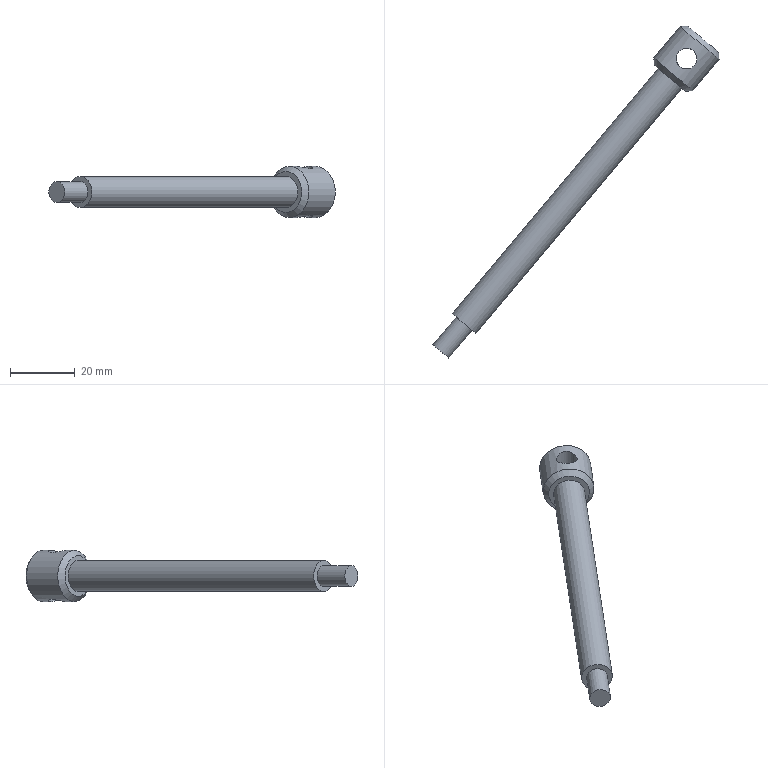Component | NX | EJE | 1 solid | 10 faces | volume 9839 mm3 | cylinder 4 | plane 4 | cone 2 | commonest cylinder face diameters 6.35 x2 15.748 x1 9.525 x1